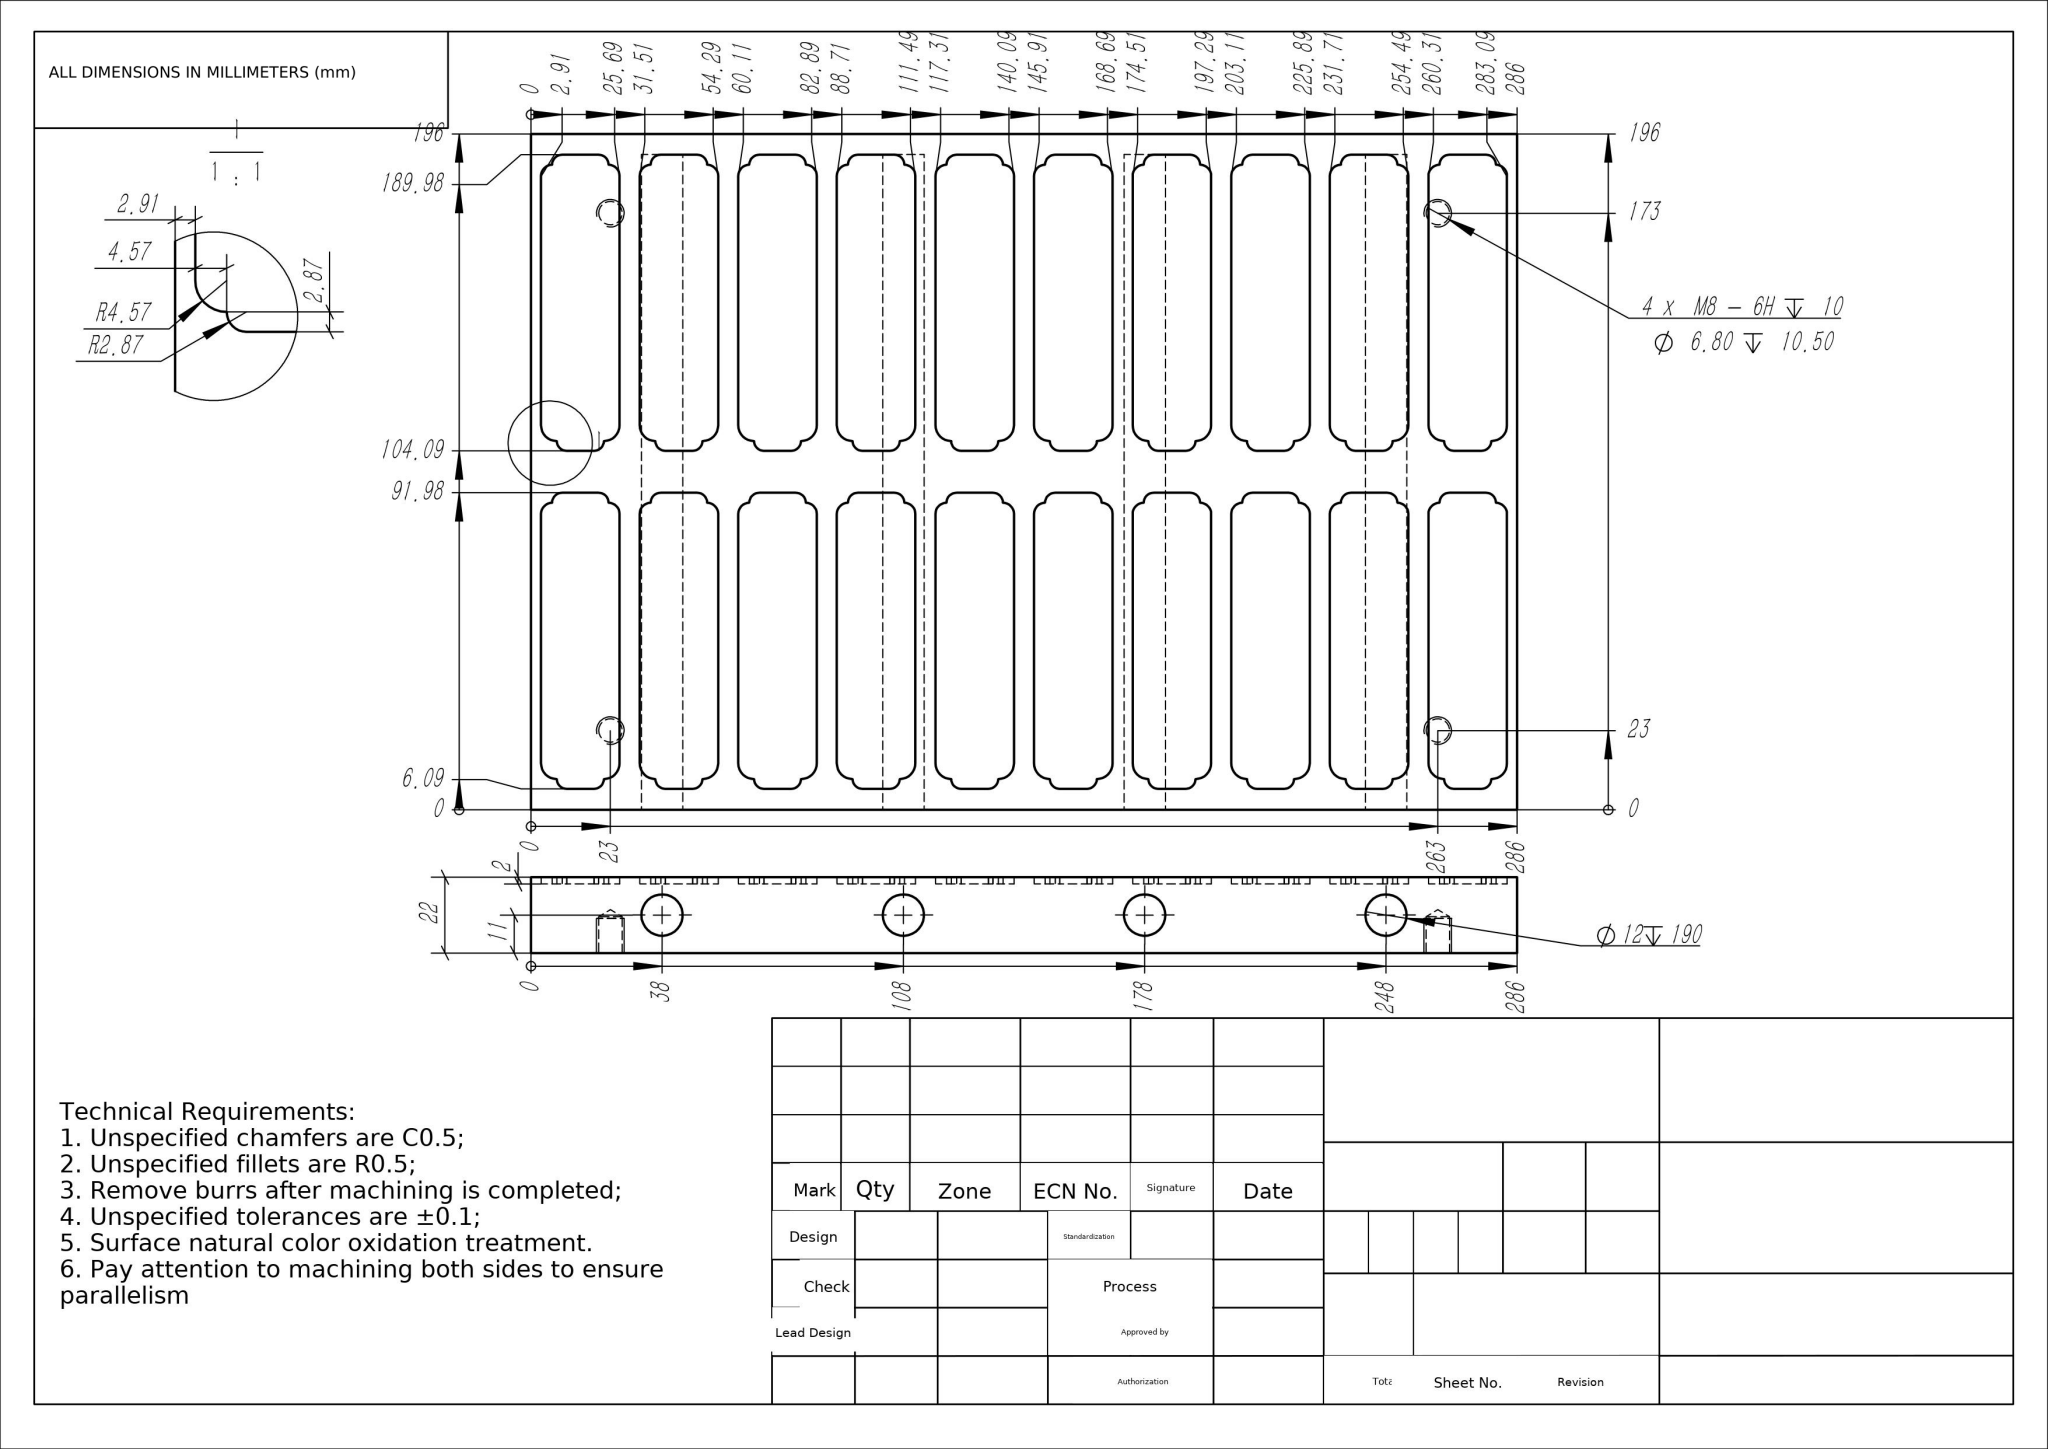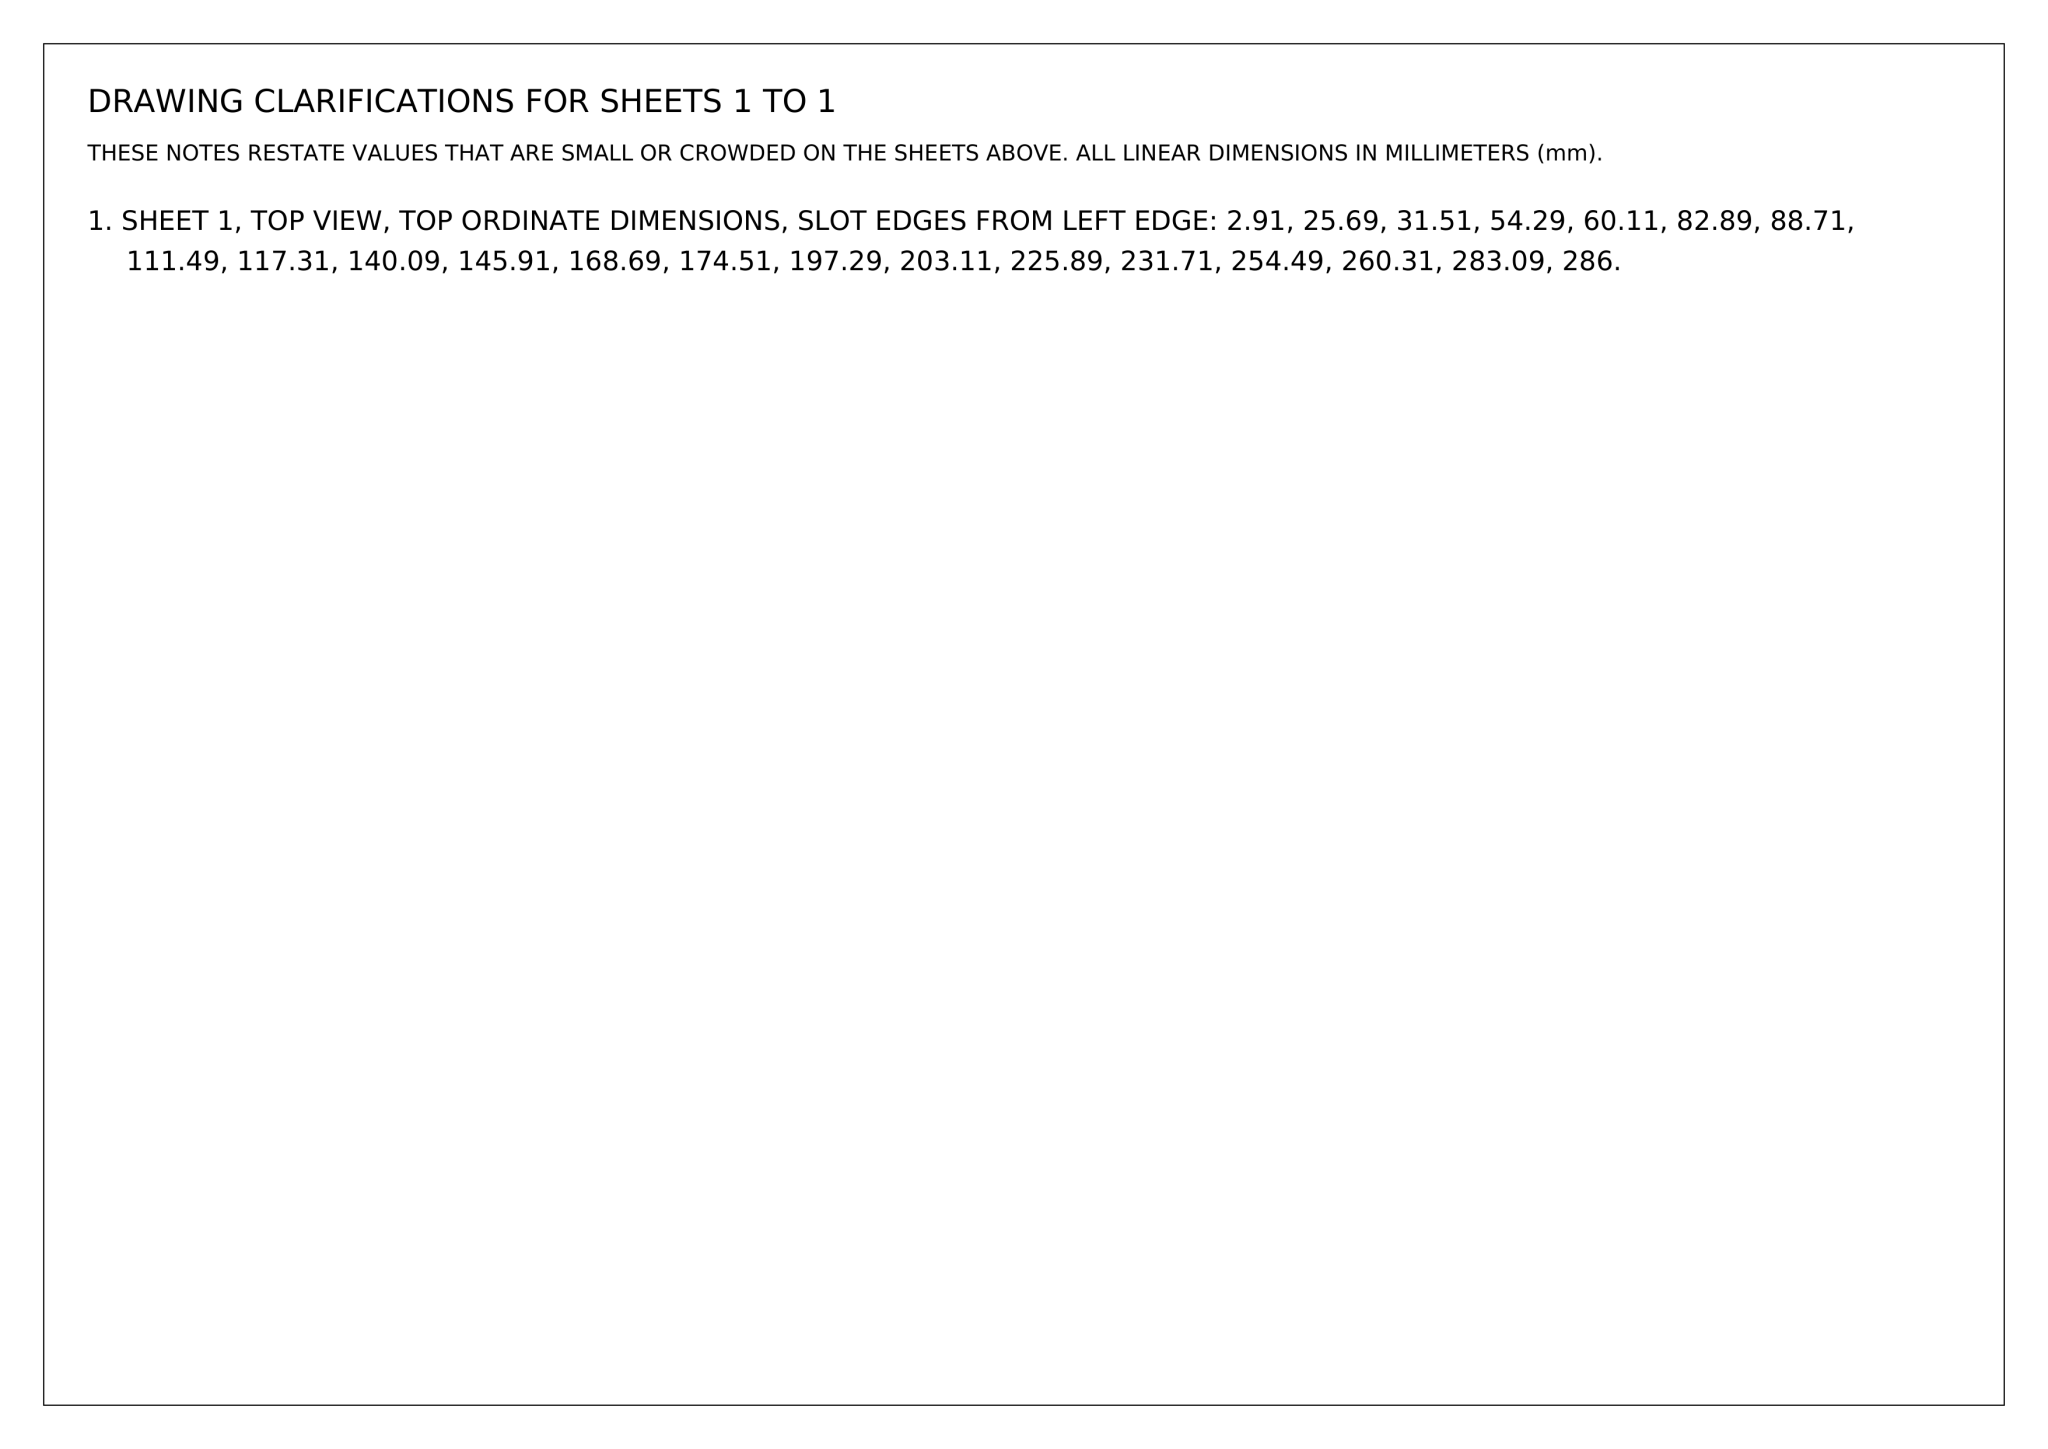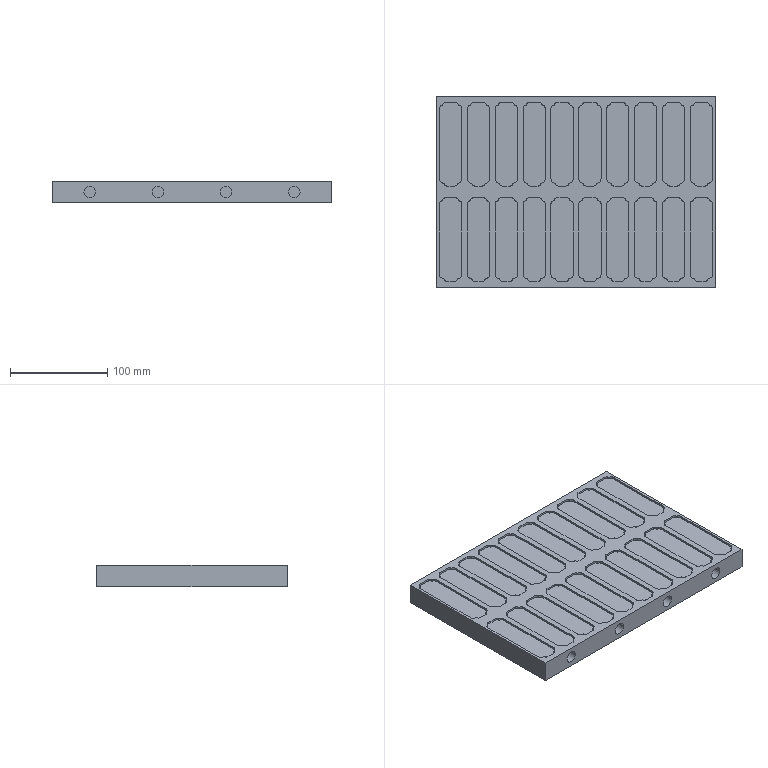Part | NX | mm | 1 solid | 294 faces | box 286 x 196 x 22 mm | volume 1070011 mm3 | cylinder 176 | plane 110 | cone 8 | commonest cylinder face diameters 5.86 x40 6.4 x40 5.74 x40 9.14 x40 12 x8 6.8 x8